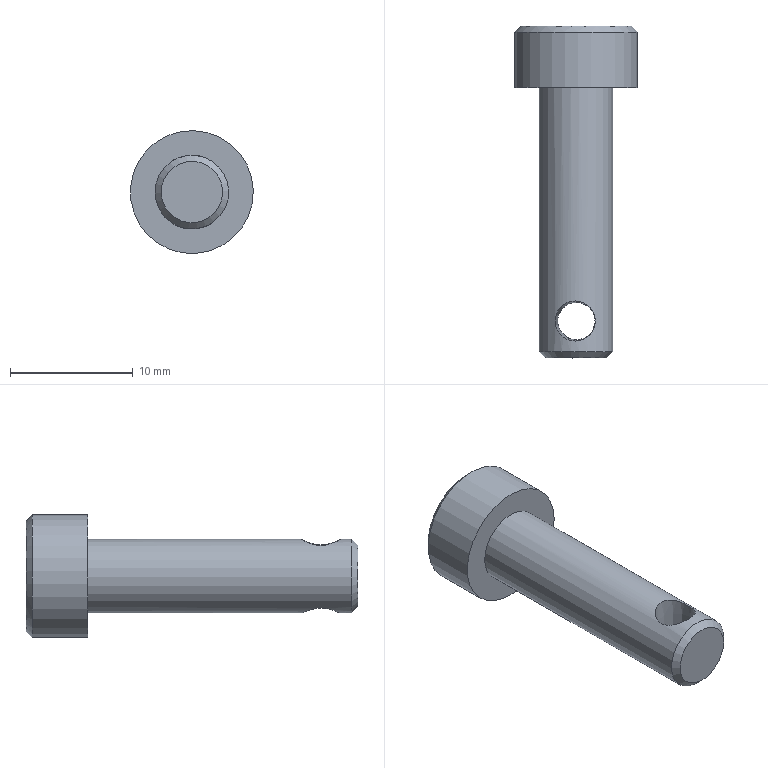Component | NX | DOWEL_PIN | 1 solid | 21 faces | volume 840 mm3 | plane 10 | cylinder 8 | cone 3 | commonest cylinder face diameters 4 x6 6 x1 10 x1